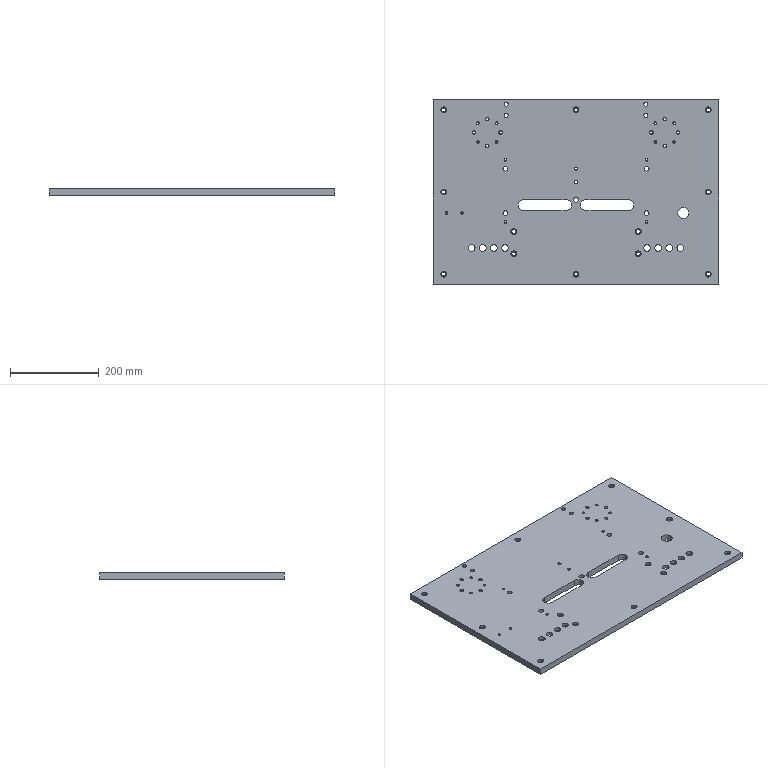Component | SolidWorks | DoubleFilmTransport-1_LongitudinalSealingPanel-1 | 1 solid | 216 faces | volume 3824377 mm3 | cylinder 144 | cone 44 | plane 28 | commonest cylinder face diameters 9 x32 5 x28 13.5 x24 6.8 x16 15 x16 11 x8 25 x8 26 x6